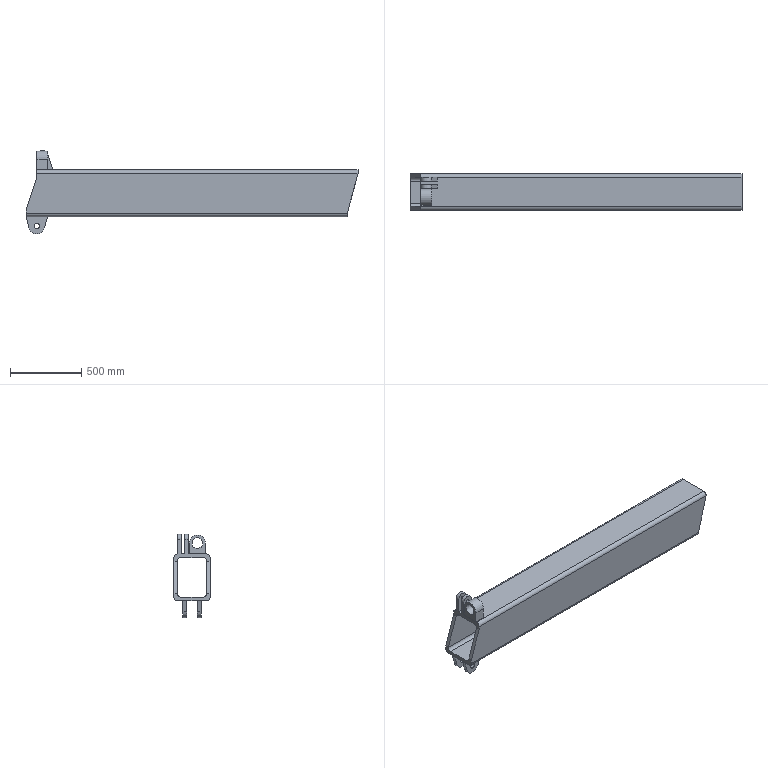Component | NX | ARM_SECTION_2 | 1 solid | 52 faces | volume 63103860 mm3 | plane 34 | cylinder 18 | commonest cylinder face diameters 50 x4 48 x4 76.2 x3 114.3 x3 25.4 x2 38 x2